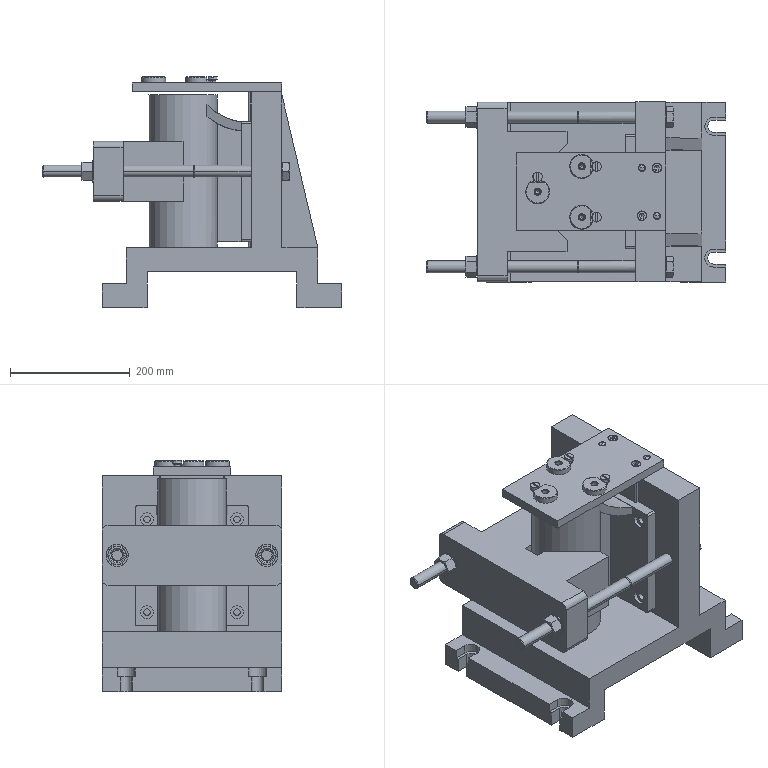Assembly | NX | mm | 20 component files | 21 solids | 461 faces | box 500 x 300 x 386 mm | volume 15579283 mm3 | plane 204 | cylinder 112 | cone 111 | torus 30 | sphere 4 | commonest cylinder face diameters 20 x22 10 x18 30 x10 10.006 x8 6 x8 37 x6 22 x6 6.8 x6
Bill of materials:
unnamed part 1 | 1 |  | Vertical hollow cylindrical tube joined by a tapered web to a rectangular side flange plate; the plate has four corner through-holes, and the tube's top end face has three small holes.
unnamed part 2 | 2 |  | Screw-like part with a cylindrical head, a hexagonal socket recess, and a stepped plain shank: a larger-diameter section under the head, then a longer smaller-diameter section.
unnamed part 3 | 2 |  | Hexagonal nut-shaped body with chamfered corners on both faces and a central round through-bore.
unnamed part 4 | 2 |  | Thin flat annular ring (plain washer shape) with a central round hole.
unnamed part 5 | 1 |  | Elongated block with rounded corners and two end through-holes; in profile it is T-shaped, with a raised central body ending in a V-shaped notch.
unnamed part 6 | 3 |  | Flanged cylindrical bushing with a central through-hole, a chamfered smaller-diameter spigot, and a straight slot cut across one side of the flange.
unnamed part 7 | 2 |  | Long slender bolt-like rod with a hexagonal head at one end and a plain cylindrical shank.
unnamed part 8 | 3 |  | Screw-like part with a slotted cylindrical head (slightly tapered sides) and a plain cylindrical shank.
unnamed part 9 | 1 |  | Angle bracket or stand: a base plate with a stepped underside and end feet, carrying a tall upright wall with a tapered back.
unnamed part 10 | 2 |  | Solid cylindrical pin with a chamfered end and a slightly domed opposite end.
unnamed part 11 | 1 |  | Flat rectangular plate with three large round through-holes, three small conical-bottom holes, and four small holes near one end, two of which have counterbored or chamfered rims.
Mates:
1. fix | jig_body 1 component
2. distance | gas_engine_bracket 1 face | jig_body 1 face
3. touch align | gas_engine_bracket 1 face | jig_body 1 face
4. touch align | gas_engine_bracket 1 face | jig_body 1 face
5. align lock | V_block 1 face | jig_body 1 face
6. align lock | V_block 1 face | jig_body 1 face
7. touch align | V_block 1 face | gas_engine_bracket 1 face
8. concentric | washer_20 2 edge | V_block 1 edge
9. concentric | washer_20 1 edge | V_block 1 edge
10. concentric | nut_M20 1 edge | washer_20 2 edge
11. concentric | nut_M20 2 edge | washer_20 1 edge
12. concentric | bolt_M20x400 2 edge | jig_body 1 edge
13. concentric | bolt_M20x400 1 edge | jig_body 1 edge
14. align lock | guide_plate 1 face | jig_body 1 face
15. concentric | guide_plate 1 edge | jig_body 1 edge
16. concentric | allen_M10x40 1 edge | guide_plate 1 edge
17. concentric | allen_M10x40 2 edge | guide_plate 1 edge
18. concentric | dowel_pin_10x60 1 edge | guide_plate 1 edge
19. concentric | dowel_pin_10x60 2 edge | guide_plate 1 edge
20. concentric | drill_bushing 3 edge | guide_plate 1 edge
21. concentric | drill_bushing 1 edge | guide_plate 1 edge
22. concentric | drill_bushing 2 edge | guide_plate 1 edge
23. align lock | M10x13_screw 2 face | guide_plate 1 face
24. align lock | M10x13_screw 1 face | guide_plate 1 face
25. align lock | M10x13_screw 3 face | guide_plate 1 face
26. touch align | M10x13_screw 2 face | drill_bushing 2 face
27. touch align | M10x13_screw 3 face | drill_bushing 1 face
28. touch align | M10x13_screw 1 face | drill_bushing 3 face